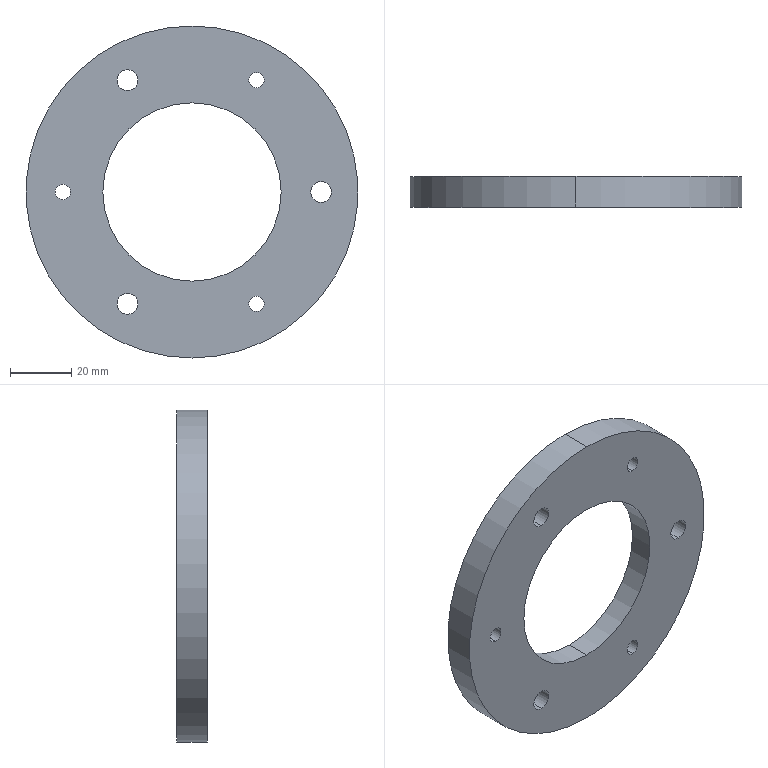Component | SolidWorks | Assembly4.1-1_115.1-1 | 1 solid | 21 faces | box 108 x 10 x 108 mm | volume 61097 mm3 | cylinder 18 | plane 3 | commonest cylinder face diameters 6.8 x6 5 x6 70 x2 108 x2 58 x2
build123d program:
from build123d import *

# Parameters (mm, degrees)
SKETCH1_R             = 54
SKETCH1_R_2           = 29
BOSS_EXTRUDE1_DEPTH   = 10
CIRPATTERN1_COUNT     = 3
SKETCH4_R             = 35
CUT_EXTRUDE1_DEPTH    = 2
M8_TAPPED_HOLE1_D     = 6.8
M8_TAPPED_HOLE1_DEPTH = 19.75
M8_TAPPED_HOLE1_TIP   = 2.043


with BuildPart() as part:
    # Sketch1 → Boss-Extrude1 (new body)
    with BuildSketch(Plane.XY):
        Circle(SKETCH1_R)
        Circle(SKETCH1_R_2, mode=Mode.SUBTRACT)
    extrude(amount=BOSS_EXTRUDE1_DEPTH)

    # Sketch2 → M6 Tapped Hole1 (revolve, cut)
    with BuildSketch(Plane(origin=(0, 42, 10), x_dir=(0, -1, 0), z_dir=(1, 0, 0))):
        Polygon((0, 0), (0, 16.502), (2.5, 15), (2.5, 0), align=None)
    m6_tapped_hole1 = revolve(axis=Axis((0, 42, 16.35), (0, 0, -1)), mode=Mode.SUBTRACT)

    # CirPattern1: M6 Tapped Hole1 ×3 about axis
    cirpattern1_axis = Axis((0, 0, 0), (0, 0, 1))
    for i in range(1, CIRPATTERN1_COUNT):
        add(m6_tapped_hole1.rotate(cirpattern1_axis, i * 360 / CIRPATTERN1_COUNT), mode=Mode.SUBTRACT)

    # Sketch4 → Cut-Extrude1 (cut)
    with BuildSketch(Plane.XY.offset(10)):
        Circle(SKETCH4_R)
    extrude(amount=-CUT_EXTRUDE1_DEPTH, mode=Mode.SUBTRACT)

    # M8 Tapped Hole1
    with Locations(Plane.XY.offset(10)):
        with Locations((36.373, 21), (-36.373, 21), (0, -42)):
            Hole(M8_TAPPED_HOLE1_D / 2, depth=M8_TAPPED_HOLE1_DEPTH)
            with Locations((0, 0, -(M8_TAPPED_HOLE1_DEPTH + M8_TAPPED_HOLE1_TIP / 2))):  # 118° drill point
                Cone(0, M8_TAPPED_HOLE1_D / 2, M8_TAPPED_HOLE1_TIP, mode=Mode.SUBTRACT)


solid = part.part

# Placed as in the assembly
solid = solid.moved(Location((0, -47.5, -0.4), (-90, 0, 90)))
STEP:
#1=COLOUR_RGB('',0.7922,0.8196,0.9333);
#2=FILL_AREA_STYLE_COLOUR('',#1);
#3=FILL_AREA_STYLE('',(#2));
#4=SURFACE_STYLE_FILL_AREA(#3);
#5=SURFACE_SIDE_STYLE('',(#4));
#6=SURFACE_STYLE_USAGE(.BOTH.,#5);
#7=PRESENTATION_STYLE_ASSIGNMENT((#6));
#8=CARTESIAN_POINT('',(-0.8268,-1.87,-1.314));
#9=VERTEX_POINT('',#8);
#10=CARTESIAN_POINT('',(-0.8268,-1.87,-1.582));
#11=VERTEX_POINT('',#10);
#12=CARTESIAN_POINT('',(-0.8268,-1.87,-1.448));
#13=DIRECTION('',(0.,1.,-0.));
#14=DIRECTION('',(0.,0.,-1.));
#15=AXIS2_PLACEMENT_3D('',#12,#13,#14);
#16=CIRCLE('',#15,0.1339);
#17=EDGE_CURVE('',#9,#11,#16,.T.);
#18=ORIENTED_EDGE('',*,*,#17,.F.);
#19=CARTESIAN_POINT('',(-0.8268,-1.476,-1.314));
#20=VERTEX_POINT('',#19);
#21=CARTESIAN_POINT('',(-0.8268,-1.476,-1.314));
#22=DIRECTION('',(0.,1.,-0.));
#23=VECTOR('',#22,39.37);
#24=LINE('',#21,#23);
#25=EDGE_CURVE('',#9,#20,#24,.T.);
#26=ORIENTED_EDGE('',*,*,#25,.T.);
#27=CARTESIAN_POINT('',(-0.8268,-1.476,-1.582));
#28=VERTEX_POINT('',#27);
#29=CARTESIAN_POINT('',(-0.8268,-1.476,-1.448));
#30=DIRECTION('',(0.,1.,-0.));
#31=DIRECTION('',(0.,0.,-1.));
#32=AXIS2_PLACEMENT_3D('',#29,#30,#31);
#33=CIRCLE('',#32,0.1339);
#34=EDGE_CURVE('',#20,#28,#33,.T.);
#35=ORIENTED_EDGE('',*,*,#34,.T.);
#36=CARTESIAN_POINT('',(-0.8268,-1.476,-1.582));
#37=DIRECTION('',(0.,1.,-0.));
#38=VECTOR('',#37,39.37);
#39=LINE('',#36,#38);
#40=EDGE_CURVE('',#11,#28,#39,.T.);
#41=ORIENTED_EDGE('',*,*,#40,.F.);
#42=EDGE_LOOP('',(#18,#26,#35,#41));
#43=FACE_OUTER_BOUND('',#42,.T.);
#44=CARTESIAN_POINT('',(-0.8268,-1.476,-1.448));
#45=DIRECTION('',(0.,1.,-0.));
#46=DIRECTION('',(0.,0.,-1.));
#47=AXIS2_PLACEMENT_3D('',#44,#45,#46);
#48=CYLINDRICAL_SURFACE('',#47,0.1339);
#49=ADVANCED_FACE('',(#43),#48,.F.);
#50=CARTESIAN_POINT('',(-0.8268,-1.87,1.55));
#51=VERTEX_POINT('',#50);
#52=CARTESIAN_POINT('',(-0.8268,-1.87,1.282));
#53=VERTEX_POINT('',#52);
#54=CARTESIAN_POINT('',(-0.8268,-1.87,1.416));
#55=DIRECTION('',(0.,1.,-0.));
#56=DIRECTION('',(0.,0.,-1.));
#57=AXIS2_PLACEMENT_3D('',#54,#55,#56);
#58=CIRCLE('',#57,0.1339);
#59=EDGE_CURVE('',#51,#53,#58,.T.);
#60=ORIENTED_EDGE('',*,*,#59,.F.);
#61=CARTESIAN_POINT('',(-0.8268,-1.476,1.55));
#62=VERTEX_POINT('',#61);
#63=CARTESIAN_POINT('',(-0.8268,-1.476,1.55));
#64=DIRECTION('',(0.,1.,-0.));
#65=VECTOR('',#64,39.37);
#66=LINE('',#63,#65);
#67=EDGE_CURVE('',#51,#62,#66,.T.);
#68=ORIENTED_EDGE('',*,*,#67,.T.);
#69=CARTESIAN_POINT('',(-0.8268,-1.476,1.282));
#70=VERTEX_POINT('',#69);
#71=CARTESIAN_POINT('',(-0.8268,-1.476,1.416));
#72=DIRECTION('',(0.,1.,-0.));
#73=DIRECTION('',(0.,0.,-1.));
#74=AXIS2_PLACEMENT_3D('',#71,#72,#73);
#75=CIRCLE('',#74,0.1339);
#76=EDGE_CURVE('',#62,#70,#75,.T.);
#77=ORIENTED_EDGE('',*,*,#76,.T.);
#78=CARTESIAN_POINT('',(-0.8268,-1.476,1.282));
#79=DIRECTION('',(0.,1.,-0.));
#80=VECTOR('',#79,39.37);
#81=LINE('',#78,#80);
#82=EDGE_CURVE('',#53,#70,#81,.T.);
#83=ORIENTED_EDGE('',*,*,#82,.F.);
#84=EDGE_LOOP('',(#60,#68,#77,#83));
#85=FACE_OUTER_BOUND('',#84,.T.);
#86=CARTESIAN_POINT('',(-0.8268,-1.476,1.416));
#87=DIRECTION('',(0.,1.,-0.));
#88=DIRECTION('',(0.,0.,-1.));
#89=AXIS2_PLACEMENT_3D('',#86,#87,#88);
#90=CYLINDRICAL_SURFACE('',#89,0.1339);
#91=ADVANCED_FACE('',(#85),#90,.F.);
#92=CARTESIAN_POINT('',(1.654,-1.87,0.1181));
#93=VERTEX_POINT('',#92);
#94=CARTESIAN_POINT('',(1.654,-1.87,-0.1496));
#95=VERTEX_POINT('',#94);
#96=CARTESIAN_POINT('',(1.654,-1.87,-0.01575));
#97=DIRECTION('',(0.,1.,-0.));
#98=DIRECTION('',(0.,0.,-1.));
#99=AXIS2_PLACEMENT_3D('',#96,#97,#98);
#100=CIRCLE('',#99,0.1339);
#101=EDGE_CURVE('',#93,#95,#100,.T.);
#102=ORIENTED_EDGE('',*,*,#101,.F.);
#103=CARTESIAN_POINT('',(1.654,-1.476,0.1181));
#104=VERTEX_POINT('',#103);
#105=CARTESIAN_POINT('',(1.654,-1.476,0.1181));
#106=DIRECTION('',(0.,1.,-0.));
#107=VECTOR('',#106,39.37);
#108=LINE('',#105,#107);
#109=EDGE_CURVE('',#93,#104,#108,.T.);
#110=ORIENTED_EDGE('',*,*,#109,.T.);
#111=CARTESIAN_POINT('',(1.654,-1.476,-0.1496));
#112=VERTEX_POINT('',#111);
#113=CARTESIAN_POINT('',(1.654,-1.476,-0.01575));
#114=DIRECTION('',(0.,1.,-0.));
#115=DIRECTION('',(0.,0.,-1.));
#116=AXIS2_PLACEMENT_3D('',#113,#114,#115);
#117=CIRCLE('',#116,0.1339);
#118=EDGE_CURVE('',#104,#112,#117,.T.);
#119=ORIENTED_EDGE('',*,*,#118,.T.);
#120=CARTESIAN_POINT('',(1.654,-1.476,-0.1496));
#121=DIRECTION('',(0.,1.,-0.));
#122=VECTOR('',#121,39.37);
#123=LINE('',#120,#122);
#124=EDGE_CURVE('',#95,#112,#123,.T.);
#125=ORIENTED_EDGE('',*,*,#124,.F.);
#126=EDGE_LOOP('',(#102,#110,#119,#125));
#127=FACE_OUTER_BOUND('',#126,.T.);
#128=CARTESIAN_POINT('',(1.654,-1.476,-0.01575));
#129=DIRECTION('',(0.,1.,-0.));
#130=DIRECTION('',(0.,0.,-1.));
#131=AXIS2_PLACEMENT_3D('',#128,#129,#130);
#132=CYLINDRICAL_SURFACE('',#131,0.1339);
#133=ADVANCED_FACE('',(#127),#132,.F.);
#134=CARTESIAN_POINT('',(-0.,-1.555,1.362));
#135=VERTEX_POINT('',#134);
#136=CARTESIAN_POINT('',(0.,-1.555,-1.394));
#137=VERTEX_POINT('',#136);
#138=CARTESIAN_POINT('',(-0.,-1.555,-0.01575));
#139=DIRECTION('',(0.,1.,-0.));
#140=DIRECTION('',(0.,0.,-1.));
#141=AXIS2_PLACEMENT_3D('',#138,#139,#140);
#142=CIRCLE('',#141,1.378);
#143=EDGE_CURVE('',#135,#137,#142,.T.);
#144=ORIENTED_EDGE('',*,*,#143,.F.);
#145=CARTESIAN_POINT('',(-0.,-1.476,1.362));
#146=VERTEX_POINT('',#145);
#147=CARTESIAN_POINT('',(-0.,-1.555,1.362));
#148=DIRECTION('',(0.,1.,-0.));
#149=VECTOR('',#148,39.37);
#150=LINE('',#147,#149);
#151=EDGE_CURVE('',#135,#146,#150,.T.);
#152=ORIENTED_EDGE('',*,*,#151,.T.);
#153=CARTESIAN_POINT('',(0.,-1.476,-1.394));
#154=VERTEX_POINT('',#153);
#155=CARTESIAN_POINT('',(-0.,-1.476,-0.01575));
#156=DIRECTION('',(0.,1.,-0.));
#157=DIRECTION('',(0.,0.,-1.));
#158=AXIS2_PLACEMENT_3D('',#155,#156,#157);
#159=CIRCLE('',#158,1.378);
#160=EDGE_CURVE('',#146,#154,#159,.T.);
#161=ORIENTED_EDGE('',*,*,#160,.T.);
#162=CARTESIAN_POINT('',(0.,-1.555,-1.394));
#163=DIRECTION('',(0.,1.,-0.));
#164=VECTOR('',#163,39.37);
#165=LINE('',#162,#164);
#166=EDGE_CURVE('',#137,#154,#165,.T.);
#167=ORIENTED_EDGE('',*,*,#166,.F.);
#168=EDGE_LOOP('',(#144,#152,#161,#167));
#169=FACE_OUTER_BOUND('',#168,.T.);
#170=CARTESIAN_POINT('',(-0.,-1.555,-0.01575));
#171=DIRECTION('',(0.,1.,-0.));
#172=DIRECTION('',(0.,0.,-1.));
#173=AXIS2_PLACEMENT_3D('',#170,#171,#172);
#174=CYLINDRICAL_SURFACE('',#173,1.378);
#175=ADVANCED_FACE('',(#169),#174,.F.);
#176=CARTESIAN_POINT('',(0.8268,-1.87,1.515));
#177=VERTEX_POINT('',#176);
#178=CARTESIAN_POINT('',(0.8268,-1.87,1.318));
#179=VERTEX_POINT('',#178);
#180=CARTESIAN_POINT('',(0.8268,-1.87,1.416));
#181=DIRECTION('',(0.,1.,-0.));
#182=DIRECTION('',(0.,0.,-1.));
#183=AXIS2_PLACEMENT_3D('',#180,#181,#182);
#184=CIRCLE('',#183,0.09843);
#185=EDGE_CURVE('',#177,#179,#184,.T.);
#186=ORIENTED_EDGE('',*,*,#185,.F.);
#187=CARTESIAN_POINT('',(0.8268,-1.476,1.515));
#188=VERTEX_POINT('',#187);
#189=CARTESIAN_POINT('',(0.8268,-1.476,1.515));
#190=DIRECTION('',(0.,1.,-0.));
#191=VECTOR('',#190,39.37);
#192=LINE('',#189,#191);
#193=EDGE_CURVE('',#177,#188,#192,.T.);
#194=ORIENTED_EDGE('',*,*,#193,.T.);
#195=CARTESIAN_POINT('',(0.8268,-1.476,1.318));
#196=VERTEX_POINT('',#195);
#197=CARTESIAN_POINT('',(0.8268,-1.476,1.416));
#198=DIRECTION('',(0.,1.,-0.));
#199=DIRECTION('',(0.,0.,-1.));
#200=AXIS2_PLACEMENT_3D('',#197,#198,#199);
#201=CIRCLE('',#200,0.09843);
#202=EDGE_CURVE('',#188,#196,#201,.T.);
#203=ORIENTED_EDGE('',*,*,#202,.T.);
#204=CARTESIAN_POINT('',(0.8268,-1.476,1.318));
#205=DIRECTION('',(0.,1.,-0.));
#206=VECTOR('',#205,39.37);
#207=LINE('',#204,#206);
#208=EDGE_CURVE('',#179,#196,#207,.T.);
#209=ORIENTED_EDGE('',*,*,#208,.F.);
#210=EDGE_LOOP('',(#186,#194,#203,#209));
#211=FACE_OUTER_BOUND('',#210,.T.);
#212=CARTESIAN_POINT('',(0.8268,-1.476,1.416));
#213=DIRECTION('',(0.,1.,-0.));
#214=DIRECTION('',(0.,0.,-1.));
#215=AXIS2_PLACEMENT_3D('',#212,#213,#214);
#216=CYLINDRICAL_SURFACE('',#215,0.09843);
#217=ADVANCED_FACE('',(#211),#216,.F.);
#218=CARTESIAN_POINT('',(0.8268,-1.87,-1.349));
#219=VERTEX_POINT('',#218);
#220=CARTESIAN_POINT('',(0.8268,-1.87,-1.546));
#221=VERTEX_POINT('',#220);
#222=CARTESIAN_POINT('',(0.8268,-1.87,-1.448));
#223=DIRECTION('',(0.,1.,-0.));
#224=DIRECTION('',(0.,0.,-1.));
#225=AXIS2_PLACEMENT_3D('',#222,#223,#224);
#226=CIRCLE('',#225,0.09843);
#227=EDGE_CURVE('',#219,#221,#226,.T.);
#228=ORIENTED_EDGE('',*,*,#227,.F.);
#229=CARTESIAN_POINT('',(0.8268,-1.476,-1.349));
#230=VERTEX_POINT('',#229);
#231=CARTESIAN_POINT('',(0.8268,-1.476,-1.349));
#232=DIRECTION('',(0.,1.,-0.));
#233=VECTOR('',#232,39.37);
#234=LINE('',#231,#233);
#235=EDGE_CURVE('',#219,#230,#234,.T.);
#236=ORIENTED_EDGE('',*,*,#235,.T.);
#237=CARTESIAN_POINT('',(0.8268,-1.476,-1.546));
#238=VERTEX_POINT('',#237);
#239=CARTESIAN_POINT('',(0.8268,-1.476,-1.448));
#240=DIRECTION('',(0.,1.,-0.));
#241=DIRECTION('',(0.,0.,-1.));
#242=AXIS2_PLACEMENT_3D('',#239,#240,#241);
#243=CIRCLE('',#242,0.09843);
#244=EDGE_CURVE('',#230,#238,#243,.T.);
#245=ORIENTED_EDGE('',*,*,#244,.T.);
#246=CARTESIAN_POINT('',(0.8268,-1.476,-1.546));
#247=DIRECTION('',(0.,1.,-0.));
#248=VECTOR('',#247,39.37);
#249=LINE('',#246,#248);
#250=EDGE_CURVE('',#221,#238,#249,.T.);
#251=ORIENTED_EDGE('',*,*,#250,.F.);
#252=EDGE_LOOP('',(#228,#236,#245,#251));
#253=FACE_OUTER_BOUND('',#252,.T.);
#254=CARTESIAN_POINT('',(0.8268,-1.476,-1.448));
#255=DIRECTION('',(0.,1.,-0.));
#256=DIRECTION('',(0.,0.,-1.));
#257=AXIS2_PLACEMENT_3D('',#254,#255,#256);
#258=CYLINDRICAL_SURFACE('',#257,0.09843);
#259=ADVANCED_FACE('',(#253),#258,.F.);
#260=CARTESIAN_POINT('',(-1.654,-1.87,0.08268));
#261=VERTEX_POINT('',#260);
#262=CARTESIAN_POINT('',(-1.654,-1.87,-0.1142));
#263=VERTEX_POINT('',#262);
#264=CARTESIAN_POINT('',(-1.654,-1.87,-0.01575));
#265=DIRECTION('',(0.,1.,-0.));
#266=DIRECTION('',(0.,0.,-1.));
#267=AXIS2_PLACEMENT_3D('',#264,#265,#266);
#268=CIRCLE('',#267,0.09843);
#269=EDGE_CURVE('',#261,#263,#268,.T.);
#270=ORIENTED_EDGE('',*,*,#269,.F.);
#271=CARTESIAN_POINT('',(-1.654,-1.476,0.08268));
#272=VERTEX_POINT('',#271);
#273=CARTESIAN_POINT('',(-1.654,-1.476,0.08268));
#274=DIRECTION('',(0.,1.,-0.));
#275=VECTOR('',#274,39.37);
#276=LINE('',#273,#275);
#277=EDGE_CURVE('',#261,#272,#276,.T.);
#278=ORIENTED_EDGE('',*,*,#277,.T.);
#279=CARTESIAN_POINT('',(-1.654,-1.476,-0.1142));
#280=VERTEX_POINT('',#279);
#281=CARTESIAN_POINT('',(-1.654,-1.476,-0.01575));
#282=DIRECTION('',(0.,1.,-0.));
#283=DIRECTION('',(0.,0.,-1.));
#284=AXIS2_PLACEMENT_3D('',#281,#282,#283);
#285=CIRCLE('',#284,0.09843);
#286=EDGE_CURVE('',#272,#280,#285,.T.);
#287=ORIENTED_EDGE('',*,*,#286,.T.);
#288=CARTESIAN_POINT('',(-1.654,-1.476,-0.1142));
#289=DIRECTION('',(0.,1.,-0.));
#290=VECTOR('',#289,39.37);
#291=LINE('',#288,#290);
#292=EDGE_CURVE('',#263,#280,#291,.T.);
#293=ORIENTED_EDGE('',*,*,#292,.F.);
#294=EDGE_LOOP('',(#270,#278,#287,#293));
#295=FACE_OUTER_BOUND('',#294,.T.);
#296=CARTESIAN_POINT('',(-1.654,-1.476,-0.01575));
#297=DIRECTION('',(0.,1.,-0.));
#298=DIRECTION('',(0.,0.,-1.));
#299=AXIS2_PLACEMENT_3D('',#296,#297,#298);
#300=CYLINDRICAL_SURFACE('',#299,0.09843);
#301=ADVANCED_FACE('',(#295),#300,.F.);
#302=CARTESIAN_POINT('',(0.,-1.476,-2.142));
#303=VERTEX_POINT('',#302);
#304=CARTESIAN_POINT('',(-0.,-1.476,2.11));
#305=VERTEX_POINT('',#304);
#306=CARTESIAN_POINT('',(-0.,-1.476,-0.01575));
#307=DIRECTION('',(0.,1.,-0.));
#308=DIRECTION('',(0.,0.,-1.));
#309=AXIS2_PLACEMENT_3D('',#306,#307,#308);
#310=CIRCLE('',#309,2.126);
#311=EDGE_CURVE('',#303,#305,#310,.T.);
#312=ORIENTED_EDGE('',*,*,#311,.F.);
#313=CARTESIAN_POINT('',(0.,-1.87,-2.142));
#314=VERTEX_POINT('',#313);
#315=CARTESIAN_POINT('',(0.,-1.476,-2.142));
#316=DIRECTION('',(-0.,-1.,0.));
#317=VECTOR('',#316,39.37);
#318=LINE('',#315,#317);
#319=EDGE_CURVE('',#303,#314,#318,.T.);
#320=ORIENTED_EDGE('',*,*,#319,.T.);
#321=CARTESIAN_POINT('',(-0.,-1.87,2.11));
#322=VERTEX_POINT('',#321);
#323=CARTESIAN_POINT('',(-0.,-1.87,-0.01575));
#324=DIRECTION('',(0.,1.,-0.));
#325=DIRECTION('',(0.,0.,-1.));
#326=AXIS2_PLACEMENT_3D('',#323,#324,#325);
#327=CIRCLE('',#326,2.126);
#328=EDGE_CURVE('',#314,#322,#327,.T.);
#329=ORIENTED_EDGE('',*,*,#328,.T.);
#330=CARTESIAN_POINT('',(-0.,-1.476,2.11));
#331=DIRECTION('',(-0.,-1.,0.));
#332=VECTOR('',#331,39.37);
#333=LINE('',#330,#332);
#334=EDGE_CURVE('',#305,#322,#333,.T.);
#335=ORIENTED_EDGE('',*,*,#334,.F.);
#336=EDGE_LOOP('',(#312,#320,#329,#335));
#337=FACE_OUTER_BOUND('',#336,.T.);
#338=CARTESIAN_POINT('',(-0.,-1.476,-0.01575));
#339=DIRECTION('',(-0.,-1.,0.));
#340=DIRECTION('',(-0.,0.,1.));
#341=AXIS2_PLACEMENT_3D('',#338,#339,#340);
#342=CYLINDRICAL_SURFACE('',#341,2.126);
#343=ADVANCED_FACE('',(#337),#342,.T.);
#344=CARTESIAN_POINT('',(-0.,-1.555,1.126));
#345=VERTEX_POINT('',#344);
#346=CARTESIAN_POINT('',(-0.,-1.555,-1.157));
#347=VERTEX_POINT('',#346);
#348=CARTESIAN_POINT('',(-0.,-1.555,-0.01575));
#349=DIRECTION('',(0.,1.,-0.));
#350=DIRECTION('',(0.,0.,-1.));
#351=AXIS2_PLACEMENT_3D('',#348,#349,#350);
#352=CIRCLE('',#351,1.142);
#353=EDGE_CURVE('',#345,#347,#352,.T.);
#354=ORIENTED_EDGE('',*,*,#353,.T.);
#355=CARTESIAN_POINT('',(-0.,-1.87,-1.157));
#356=VERTEX_POINT('',#355);
#357=CARTESIAN_POINT('',(-0.,-1.476,-1.157));
#358=DIRECTION('',(-0.,-1.,0.));
#359=VECTOR('',#358,39.37);
#360=LINE('',#357,#359);
#361=EDGE_CURVE('',#347,#356,#360,.T.);
#362=ORIENTED_EDGE('',*,*,#361,.T.);
#363=CARTESIAN_POINT('',(-0.,-1.87,1.126));
#364=VERTEX_POINT('',#363);
#365=CARTESIAN_POINT('',(-0.,-1.87,-0.01575));
#366=DIRECTION('',(0.,1.,-0.));
#367=DIRECTION('',(0.,0.,-1.));
#368=AXIS2_PLACEMENT_3D('',#365,#366,#367);
#369=CIRCLE('',#368,1.142);
#370=EDGE_CURVE('',#364,#356,#369,.T.);
#371=ORIENTED_EDGE('',*,*,#370,.F.);
#372=CARTESIAN_POINT('',(-0.,-1.476,1.126));
#373=DIRECTION('',(-0.,-1.,0.));
#374=VECTOR('',#373,39.37);
#375=LINE('',#372,#374);
#376=EDGE_CURVE('',#345,#364,#375,.T.);
#377=ORIENTED_EDGE('',*,*,#376,.F.);
#378=EDGE_LOOP('',(#354,#362,#371,#377));
#379=FACE_OUTER_BOUND('',#378,.T.);
#380=CARTESIAN_POINT('',(-0.,-1.476,-0.01575));
#381=DIRECTION('',(-0.,-1.,0.));
#382=DIRECTION('',(-0.,0.,1.));
#383=AXIS2_PLACEMENT_3D('',#380,#381,#382);
#384=CYLINDRICAL_SURFACE('',#383,1.142);
#385=ADVANCED_FACE('',(#379),#384,.F.);
#386=ORIENTED_EDGE('',*,*,#361,.F.);
#387=CARTESIAN_POINT('',(-0.,-1.555,-0.01575));
#388=DIRECTION('',(0.,1.,-0.));
#389=DIRECTION('',(0.,0.,-1.));
#390=AXIS2_PLACEMENT_3D('',#387,#388,#389);
#391=CIRCLE('',#390,1.142);
#392=EDGE_CURVE('',#347,#345,#391,.T.);
#393=ORIENTED_EDGE('',*,*,#392,.T.);
#394=ORIENTED_EDGE('',*,*,#376,.T.);
#395=CARTESIAN_POINT('',(-0.,-1.87,-0.01575));
#396=DIRECTION('',(0.,1.,-0.));
#397=DIRECTION('',(0.,0.,-1.));
#398=AXIS2_PLACEMENT_3D('',#395,#396,#397);
#399=CIRCLE('',#398,1.142);
#400=EDGE_CURVE('',#356,#364,#399,.T.);
#401=ORIENTED_EDGE('',*,*,#400,.F.);
#402=EDGE_LOOP('',(#386,#393,#394,#401));
#403=FACE_OUTER_BOUND('',#402,.T.);
#404=CARTESIAN_POINT('',(-0.,-1.476,-0.01575));
#405=DIRECTION('',(-0.,-1.,0.));
#406=DIRECTION('',(-0.,0.,1.));
#407=AXIS2_PLACEMENT_3D('',#404,#405,#406);
#408=CYLINDRICAL_SURFACE('',#407,1.142);
#409=ADVANCED_FACE('',(#403),#408,.F.);
#410=CARTESIAN_POINT('',(-0.8268,-1.476,-1.448));
#411=DIRECTION('',(0.,1.,-0.));
#412=DIRECTION('',(0.,0.,-1.));
#413=AXIS2_PLACEMENT_3D('',#410,#411,#412);
#414=CIRCLE('',#413,0.1339);
#415=EDGE_CURVE('',#28,#20,#414,.T.);
#416=ORIENTED_EDGE('',*,*,#415,.F.);
#417=ORIENTED_EDGE('',*,*,#34,.F.);
#418=EDGE_LOOP('',(#416,#417));
#419=FACE_BOUND('',#418,.T.);
#420=CARTESIAN_POINT('',(-0.8268,-1.476,1.416));
#421=DIRECTION('',(0.,1.,-0.));
#422=DIRECTION('',(0.,0.,-1.));
#423=AXIS2_PLACEMENT_3D('',#420,#421,#422);
#424=CIRCLE('',#423,0.1339);
#425=EDGE_CURVE('',#70,#62,#424,.T.);
#426=ORIENTED_EDGE('',*,*,#425,.F.);
#427=ORIENTED_EDGE('',*,*,#76,.F.);
#428=EDGE_LOOP('',(#426,#427));
#429=FACE_BOUND('',#428,.T.);
#430=CARTESIAN_POINT('',(1.654,-1.476,-0.01575));
#431=DIRECTION('',(0.,1.,-0.));
#432=DIRECTION('',(0.,0.,-1.));
#433=AXIS2_PLACEMENT_3D('',#430,#431,#432);
#434=CIRCLE('',#433,0.1339);
#435=EDGE_CURVE('',#112,#104,#434,.T.);
#436=ORIENTED_EDGE('',*,*,#435,.F.);
#437=ORIENTED_EDGE('',*,*,#118,.F.);
#438=EDGE_LOOP('',(#436,#437));
#439=FACE_BOUND('',#438,.T.);
#440=CARTESIAN_POINT('',(-0.,-1.476,-0.01575));
#441=DIRECTION('',(0.,1.,-0.));
#442=DIRECTION('',(0.,0.,-1.));
#443=AXIS2_PLACEMENT_3D('',#440,#441,#442);
#444=CIRCLE('',#443,1.378);
#445=EDGE_CURVE('',#154,#146,#444,.T.);
#446=ORIENTED_EDGE('',*,*,#445,.F.);
#447=ORIENTED_EDGE('',*,*,#160,.F.);
#448=EDGE_LOOP('',(#446,#447));
#449=FACE_BOUND('',#448,.T.);
#450=CARTESIAN_POINT('',(0.8268,-1.476,1.416));
#451=DIRECTION('',(0.,1.,-0.));
#452=DIRECTION('',(0.,0.,-1.));
#453=AXIS2_PLACEMENT_3D('',#450,#451,#452);
#454=CIRCLE('',#453,0.09843);
#455=EDGE_CURVE('',#196,#188,#454,.T.);
#456=ORIENTED_EDGE('',*,*,#455,.F.);
#457=ORIENTED_EDGE('',*,*,#202,.F.);
#458=EDGE_LOOP('',(#456,#457));
#459=FACE_BOUND('',#458,.T.);
#460=CARTESIAN_POINT('',(0.8268,-1.476,-1.448));
#461=DIRECTION('',(0.,1.,-0.));
#462=DIRECTION('',(0.,0.,-1.));
#463=AXIS2_PLACEMENT_3D('',#460,#461,#462);
#464=CIRCLE('',#463,0.09843);
#465=EDGE_CURVE('',#238,#230,#464,.T.);
#466=ORIENTED_EDGE('',*,*,#465,.F.);
#467=ORIENTED_EDGE('',*,*,#244,.F.);
#468=EDGE_LOOP('',(#466,#467));
#469=FACE_BOUND('',#468,.T.);
#470=CARTESIAN_POINT('',(-1.654,-1.476,-0.01575));
#471=DIRECTION('',(0.,1.,-0.));
#472=DIRECTION('',(0.,0.,-1.));
#473=AXIS2_PLACEMENT_3D('',#470,#471,#472);
#474=CIRCLE('',#473,0.09843);
#475=EDGE_CURVE('',#280,#272,#474,.T.);
#476=ORIENTED_EDGE('',*,*,#475,.F.);
#477=ORIENTED_EDGE('',*,*,#286,.F.);
#478=EDGE_LOOP('',(#476,#477));
#479=FACE_BOUND('',#478,.T.);
#480=CARTESIAN_POINT('',(-0.,-1.476,-0.01575));
#481=DIRECTION('',(0.,1.,-0.));
#482=DIRECTION('',(0.,0.,-1.));
#483=AXIS2_PLACEMENT_3D('',#480,#481,#482);
#484=CIRCLE('',#483,2.126);
#485=EDGE_CURVE('',#305,#303,#484,.T.);
#486=ORIENTED_EDGE('',*,*,#485,.T.);
#487=ORIENTED_EDGE('',*,*,#311,.T.);
#488=EDGE_LOOP('',(#486,#487));
#489=FACE_OUTER_BOUND('',#488,.T.);
#490=CARTESIAN_POINT('',(-0.,-1.476,-0.01575));
#491=DIRECTION('',(0.,1.,-0.));
#492=DIRECTION('',(0.,-0.,-1.));
#493=AXIS2_PLACEMENT_3D('',#490,#491,#492);
#494=PLANE('',#493);
#495=ADVANCED_FACE('',(#419,#429,#439,#449,#459,#469,#479,#489),#494,.T.);
#496=CARTESIAN_POINT('',(-0.8268,-1.87,-1.448));
#497=DIRECTION('',(0.,1.,-0.));
#498=DIRECTION('',(0.,0.,-1.));
#499=AXIS2_PLACEMENT_3D('',#496,#497,#498);
#500=CIRCLE('',#499,0.1339);
#501=EDGE_CURVE('',#11,#9,#500,.T.);
#502=ORIENTED_EDGE('',*,*,#501,.T.);
#503=ORIENTED_EDGE('',*,*,#17,.T.);
#504=EDGE_LOOP('',(#502,#503));
#505=FACE_BOUND('',#504,.T.);
#506=CARTESIAN_POINT('',(-0.8268,-1.87,1.416));
#507=DIRECTION('',(0.,1.,-0.));
#508=DIRECTION('',(0.,0.,-1.));
#509=AXIS2_PLACEMENT_3D('',#506,#507,#508);
#510=CIRCLE('',#509,0.1339);
#511=EDGE_CURVE('',#53,#51,#510,.T.);
#512=ORIENTED_EDGE('',*,*,#511,.T.);
#513=ORIENTED_EDGE('',*,*,#59,.T.);
#514=EDGE_LOOP('',(#512,#513));
#515=FACE_BOUND('',#514,.T.);
#516=CARTESIAN_POINT('',(1.654,-1.87,-0.01575));
#517=DIRECTION('',(0.,1.,-0.));
#518=DIRECTION('',(0.,0.,-1.));
#519=AXIS2_PLACEMENT_3D('',#516,#517,#518);
#520=CIRCLE('',#519,0.1339);
#521=EDGE_CURVE('',#95,#93,#520,.T.);
#522=ORIENTED_EDGE('',*,*,#521,.T.);
#523=ORIENTED_EDGE('',*,*,#101,.T.);
#524=EDGE_LOOP('',(#522,#523));
#525=FACE_BOUND('',#524,.T.);
#526=CARTESIAN_POINT('',(0.8268,-1.87,1.416));
#527=DIRECTION('',(0.,1.,-0.));
#528=DIRECTION('',(0.,0.,-1.));
#529=AXIS2_PLACEMENT_3D('',#526,#527,#528);
#530=CIRCLE('',#529,0.09843);
#531=EDGE_CURVE('',#179,#177,#530,.T.);
#532=ORIENTED_EDGE('',*,*,#531,.T.);
#533=ORIENTED_EDGE('',*,*,#185,.T.);
#534=EDGE_LOOP('',(#532,#533));
#535=FACE_BOUND('',#534,.T.);
#536=CARTESIAN_POINT('',(0.8268,-1.87,-1.448));
#537=DIRECTION('',(0.,1.,-0.));
#538=DIRECTION('',(0.,0.,-1.));
#539=AXIS2_PLACEMENT_3D('',#536,#537,#538);
#540=CIRCLE('',#539,0.09843);
#541=EDGE_CURVE('',#221,#219,#540,.T.);
#542=ORIENTED_EDGE('',*,*,#541,.T.);
#543=ORIENTED_EDGE('',*,*,#227,.T.);
#544=EDGE_LOOP('',(#542,#543));
#545=FACE_BOUND('',#544,.T.);
#546=CARTESIAN_POINT('',(-1.654,-1.87,-0.01575));
#547=DIRECTION('',(0.,1.,-0.));
#548=DIRECTION('',(0.,0.,-1.));
#549=AXIS2_PLACEMENT_3D('',#546,#547,#548);
#550=CIRCLE('',#549,0.09843);
#551=EDGE_CURVE('',#263,#261,#550,.T.);
#552=ORIENTED_EDGE('',*,*,#551,.T.);
#553=ORIENTED_EDGE('',*,*,#269,.T.);
#554=EDGE_LOOP('',(#552,#553));
#555=FACE_BOUND('',#554,.T.);
#556=CARTESIAN_POINT('',(-0.,-1.87,-0.01575));
#557=DIRECTION('',(0.,1.,-0.));
#558=DIRECTION('',(0.,0.,-1.));
#559=AXIS2_PLACEMENT_3D('',#556,#557,#558);
#560=CIRCLE('',#559,2.126);
#561=EDGE_CURVE('',#322,#314,#560,.T.);
#562=ORIENTED_EDGE('',*,*,#561,.F.);
#563=ORIENTED_EDGE('',*,*,#328,.F.);
#564=EDGE_LOOP('',(#562,#563));
#565=FACE_OUTER_BOUND('',#564,.T.);
#566=ORIENTED_EDGE('',*,*,#370,.T.);
#567=ORIENTED_EDGE('',*,*,#400,.T.);
#568=EDGE_LOOP('',(#566,#567));
#569=FACE_BOUND('',#568,.T.);
#570=CARTESIAN_POINT('',(-0.,-1.87,-0.01575));
#571=DIRECTION('',(0.,1.,-0.));
#572=DIRECTION('',(0.,-0.,-1.));
#573=AXIS2_PLACEMENT_3D('',#570,#571,#572);
#574=PLANE('',#573);
#575=ADVANCED_FACE('',(#505,#515,#525,#535,#545,#555,#565,#569),#574,.F.);
#576=ORIENTED_EDGE('',*,*,#319,.F.);
#577=ORIENTED_EDGE('',*,*,#485,.F.);
#578=ORIENTED_EDGE('',*,*,#334,.T.);
#579=ORIENTED_EDGE('',*,*,#561,.T.);
#580=EDGE_LOOP('',(#576,#577,#578,#579));
#581=FACE_OUTER_BOUND('',#580,.T.);
#582=CARTESIAN_POINT('',(-0.,-1.476,-0.01575));
#583=DIRECTION('',(-0.,-1.,0.));
#584=DIRECTION('',(-0.,0.,1.));
#585=AXIS2_PLACEMENT_3D('',#582,#583,#584);
#586=CYLINDRICAL_SURFACE('',#585,2.126);
#587=ADVANCED_FACE('',(#581),#586,.T.);
#588=ORIENTED_EDGE('',*,*,#277,.F.);
#589=ORIENTED_EDGE('',*,*,#551,.F.);
#590=ORIENTED_EDGE('',*,*,#292,.T.);
#591=ORIENTED_EDGE('',*,*,#475,.T.);
#592=EDGE_LOOP('',(#588,#589,#590,#591));
#593=FACE_OUTER_BOUND('',#592,.T.);
#594=CARTESIAN_POINT('',(-1.654,-1.476,-0.01575));
#595=DIRECTION('',(0.,1.,-0.));
#596=DIRECTION('',(0.,0.,-1.));
#597=AXIS2_PLACEMENT_3D('',#594,#595,#596);
#598=CYLINDRICAL_SURFACE('',#597,0.09843);
#599=ADVANCED_FACE('',(#593),#598,.F.);
#600=ORIENTED_EDGE('',*,*,#235,.F.);
#601=ORIENTED_EDGE('',*,*,#541,.F.);
#602=ORIENTED_EDGE('',*,*,#250,.T.);
#603=ORIENTED_EDGE('',*,*,#465,.T.);
#604=EDGE_LOOP('',(#600,#601,#602,#603));
#605=FACE_OUTER_BOUND('',#604,.T.);
#606=CARTESIAN_POINT('',(0.8268,-1.476,-1.448));
#607=DIRECTION('',(0.,1.,-0.));
#608=DIRECTION('',(0.,0.,-1.));
#609=AXIS2_PLACEMENT_3D('',#606,#607,#608);
#610=CYLINDRICAL_SURFACE('',#609,0.09843);
#611=ADVANCED_FACE('',(#605),#610,.F.);
#612=ORIENTED_EDGE('',*,*,#193,.F.);
#613=ORIENTED_EDGE('',*,*,#531,.F.);
#614=ORIENTED_EDGE('',*,*,#208,.T.);
#615=ORIENTED_EDGE('',*,*,#455,.T.);
#616=EDGE_LOOP('',(#612,#613,#614,#615));
#617=FACE_OUTER_BOUND('',#616,.T.);
#618=CARTESIAN_POINT('',(0.8268,-1.476,1.416));
#619=DIRECTION('',(0.,1.,-0.));
#620=DIRECTION('',(0.,0.,-1.));
#621=AXIS2_PLACEMENT_3D('',#618,#619,#620);
#622=CYLINDRICAL_SURFACE('',#621,0.09843);
#623=ADVANCED_FACE('',(#617),#622,.F.);
#624=ORIENTED_EDGE('',*,*,#151,.F.);
#625=CARTESIAN_POINT('',(-0.,-1.555,-0.01575));
#626=DIRECTION('',(0.,1.,-0.));
#627=DIRECTION('',(0.,0.,-1.));
#628=AXIS2_PLACEMENT_3D('',#625,#626,#627);
#629=CIRCLE('',#628,1.378);
#630=EDGE_CURVE('',#137,#135,#629,.T.);
#631=ORIENTED_EDGE('',*,*,#630,.F.);
#632=ORIENTED_EDGE('',*,*,#166,.T.);
#633=ORIENTED_EDGE('',*,*,#445,.T.);
#634=EDGE_LOOP('',(#624,#631,#632,#633));
#635=FACE_OUTER_BOUND('',#634,.T.);
#636=CARTESIAN_POINT('',(-0.,-1.555,-0.01575));
#637=DIRECTION('',(0.,1.,-0.));
#638=DIRECTION('',(0.,0.,-1.));
#639=AXIS2_PLACEMENT_3D('',#636,#637,#638);
#640=CYLINDRICAL_SURFACE('',#639,1.378);
#641=ADVANCED_FACE('',(#635),#640,.F.);
#642=ORIENTED_EDGE('',*,*,#353,.F.);
#643=ORIENTED_EDGE('',*,*,#392,.F.);
#644=EDGE_LOOP('',(#642,#643));
#645=FACE_BOUND('',#644,.T.);
#646=ORIENTED_EDGE('',*,*,#630,.T.);
#647=ORIENTED_EDGE('',*,*,#143,.T.);
#648=EDGE_LOOP('',(#646,#647));
#649=FACE_OUTER_BOUND('',#648,.T.);
#650=CARTESIAN_POINT('',(-0.,-1.555,-0.01575));
#651=DIRECTION('',(0.,1.,-0.));
#652=DIRECTION('',(0.,-0.,-1.));
#653=AXIS2_PLACEMENT_3D('',#650,#651,#652);
#654=PLANE('',#653);
#655=ADVANCED_FACE('',(#645,#649),#654,.T.);
#656=ORIENTED_EDGE('',*,*,#109,.F.);
#657=ORIENTED_EDGE('',*,*,#521,.F.);
#658=ORIENTED_EDGE('',*,*,#124,.T.);
#659=ORIENTED_EDGE('',*,*,#435,.T.);
#660=EDGE_LOOP('',(#656,#657,#658,#659));
#661=FACE_OUTER_BOUND('',#660,.T.);
#662=CARTESIAN_POINT('',(1.654,-1.476,-0.01575));
#663=DIRECTION('',(0.,1.,-0.));
#664=DIRECTION('',(0.,0.,-1.));
#665=AXIS2_PLACEMENT_3D('',#662,#663,#664);
#666=CYLINDRICAL_SURFACE('',#665,0.1339);
#667=ADVANCED_FACE('',(#661),#666,.F.);
#668=ORIENTED_EDGE('',*,*,#67,.F.);
#669=ORIENTED_EDGE('',*,*,#511,.F.);
#670=ORIENTED_EDGE('',*,*,#82,.T.);
#671=ORIENTED_EDGE('',*,*,#425,.T.);
#672=EDGE_LOOP('',(#668,#669,#670,#671));
#673=FACE_OUTER_BOUND('',#672,.T.);
#674=CARTESIAN_POINT('',(-0.8268,-1.476,1.416));
#675=DIRECTION('',(0.,1.,-0.));
#676=DIRECTION('',(0.,0.,-1.));
#677=AXIS2_PLACEMENT_3D('',#674,#675,#676);
#678=CYLINDRICAL_SURFACE('',#677,0.1339);
#679=ADVANCED_FACE('',(#673),#678,.F.);
#680=ORIENTED_EDGE('',*,*,#25,.F.);
#681=ORIENTED_EDGE('',*,*,#501,.F.);
#682=ORIENTED_EDGE('',*,*,#40,.T.);
#683=ORIENTED_EDGE('',*,*,#415,.T.);
#684=EDGE_LOOP('',(#680,#681,#682,#683));
#685=FACE_OUTER_BOUND('',#684,.T.);
#686=CARTESIAN_POINT('',(-0.8268,-1.476,-1.448));
#687=DIRECTION('',(0.,1.,-0.));
#688=DIRECTION('',(0.,0.,-1.));
#689=AXIS2_PLACEMENT_3D('',#686,#687,#688);
#690=CYLINDRICAL_SURFACE('',#689,0.1339);
#691=ADVANCED_FACE('',(#685),#690,.F.);
#692=CLOSED_SHELL('',(#49,#91,#133,#175,#217,#259,#301,#343,#385,#409,#495,#575,#587,#599,#611,#623,#641,#655,#667,#679,#691));
#693=MANIFOLD_SOLID_BREP('',#692);
#694=STYLED_ITEM('',(#7),#693);
#695=(LENGTH_UNIT()NAMED_UNIT(*)SI_UNIT($,.METRE.));
#696=LENGTH_MEASURE_WITH_UNIT(LENGTH_MEASURE(0.0254),#695);
#697=DIMENSIONAL_EXPONENTS(1.,0.,0.,0.,0.,0.,0.);
#698=(CONVERSION_BASED_UNIT('',#696)LENGTH_UNIT()NAMED_UNIT(#697));
#699=UNCERTAINTY_MEASURE_WITH_UNIT(LENGTH_MEASURE(0.00001),#698,'','');
#700=(NAMED_UNIT(*)PLANE_ANGLE_UNIT()SI_UNIT($,.RADIAN.));
#701=(NAMED_UNIT(*)SI_UNIT($,.STERADIAN.)SOLID_ANGLE_UNIT());
#702=(GEOMETRIC_REPRESENTATION_CONTEXT(3)GLOBAL_UNCERTAINTY_ASSIGNED_CONTEXT((#699))GLOBAL_UNIT_ASSIGNED_CONTEXT((#698,#700,#701))REPRESENTATION_CONTEXT('',''));
#703=MECHANICAL_DESIGN_GEOMETRIC_PRESENTATION_REPRESENTATION('',(#694),#702);
#704=PRESENTATION_LAYER_ASSIGNMENT('','',(#694));
#705=CARTESIAN_POINT('',(0.,0.,0.));
#706=DIRECTION('',(0.,0.,1.));
#707=DIRECTION('',(1.,0.,0.));
#708=AXIS2_PLACEMENT_3D('',#705,#706,#707);
#709=(LENGTH_UNIT()NAMED_UNIT(*)SI_UNIT($,.METRE.));
#710=LENGTH_MEASURE_WITH_UNIT(LENGTH_MEASURE(0.0254),#709);
#711=DIMENSIONAL_EXPONENTS(1.,0.,0.,0.,0.,0.,0.);
#712=(CONVERSION_BASED_UNIT('',#710)LENGTH_UNIT()NAMED_UNIT(#711));
#713=UNCERTAINTY_MEASURE_WITH_UNIT(LENGTH_MEASURE(0.00001),#712,'','');
#714=(NAMED_UNIT(*)PLANE_ANGLE_UNIT()SI_UNIT($,.RADIAN.));
#715=(NAMED_UNIT(*)SI_UNIT($,.STERADIAN.)SOLID_ANGLE_UNIT());
#716=(GEOMETRIC_REPRESENTATION_CONTEXT(3)GLOBAL_UNCERTAINTY_ASSIGNED_CONTEXT((#713))GLOBAL_UNIT_ASSIGNED_CONTEXT((#712,#714,#715))REPRESENTATION_CONTEXT('',''));
#717=ADVANCED_BREP_SHAPE_REPRESENTATION('',(#693,#708),#716);